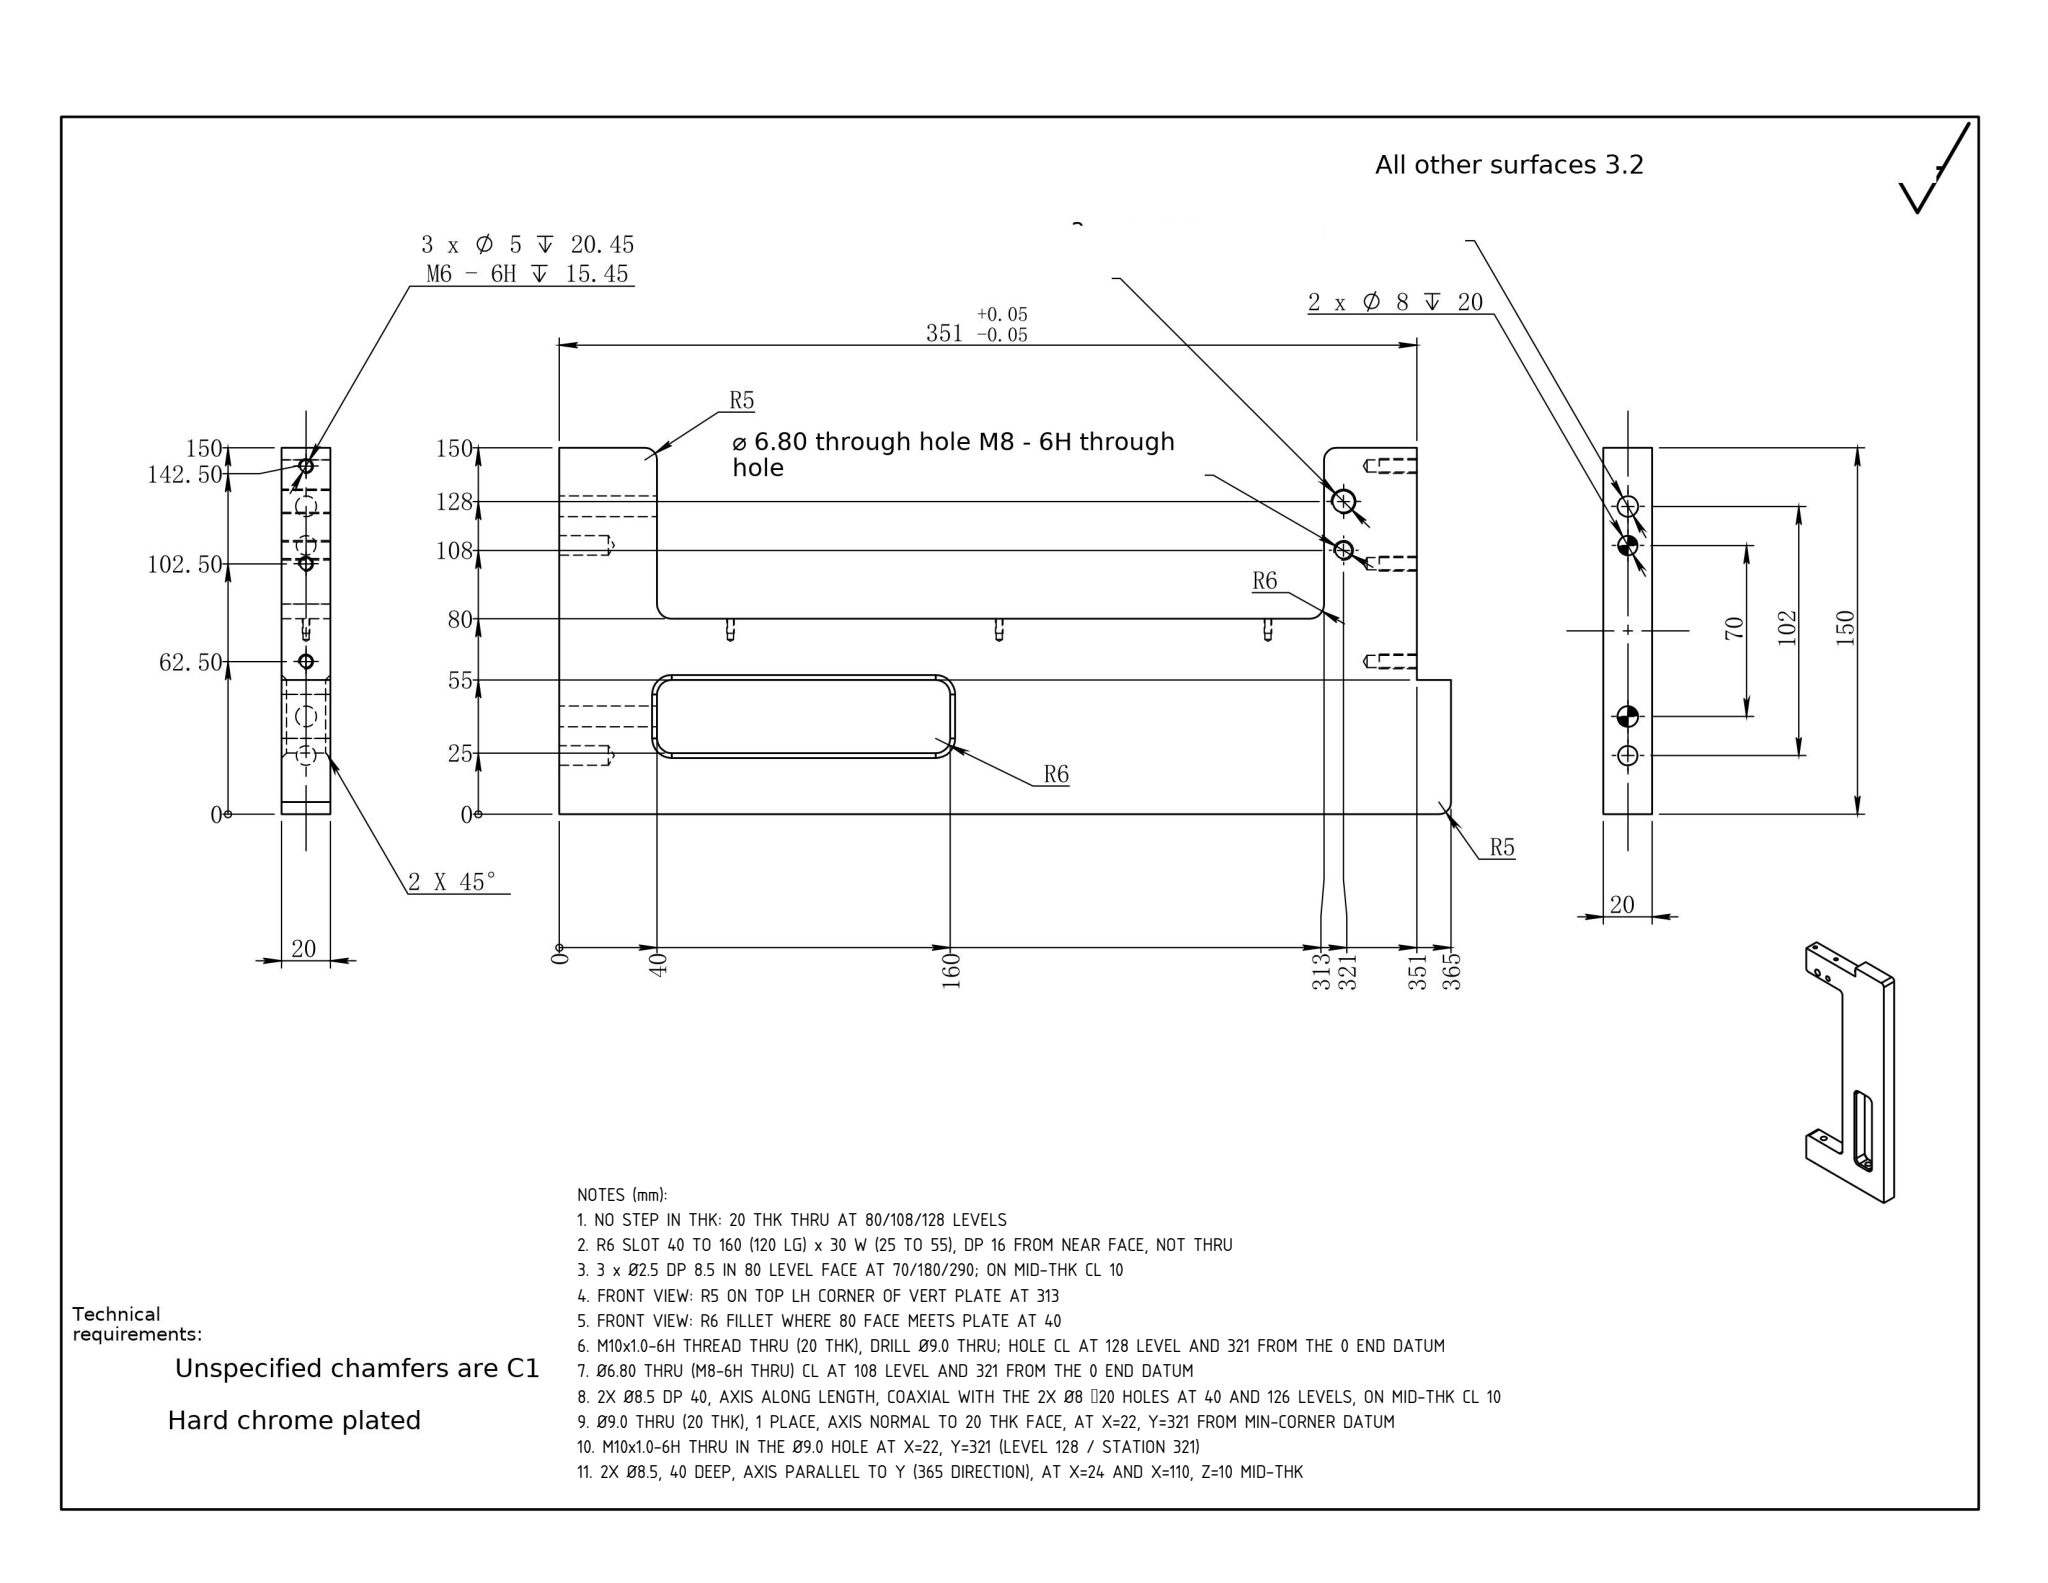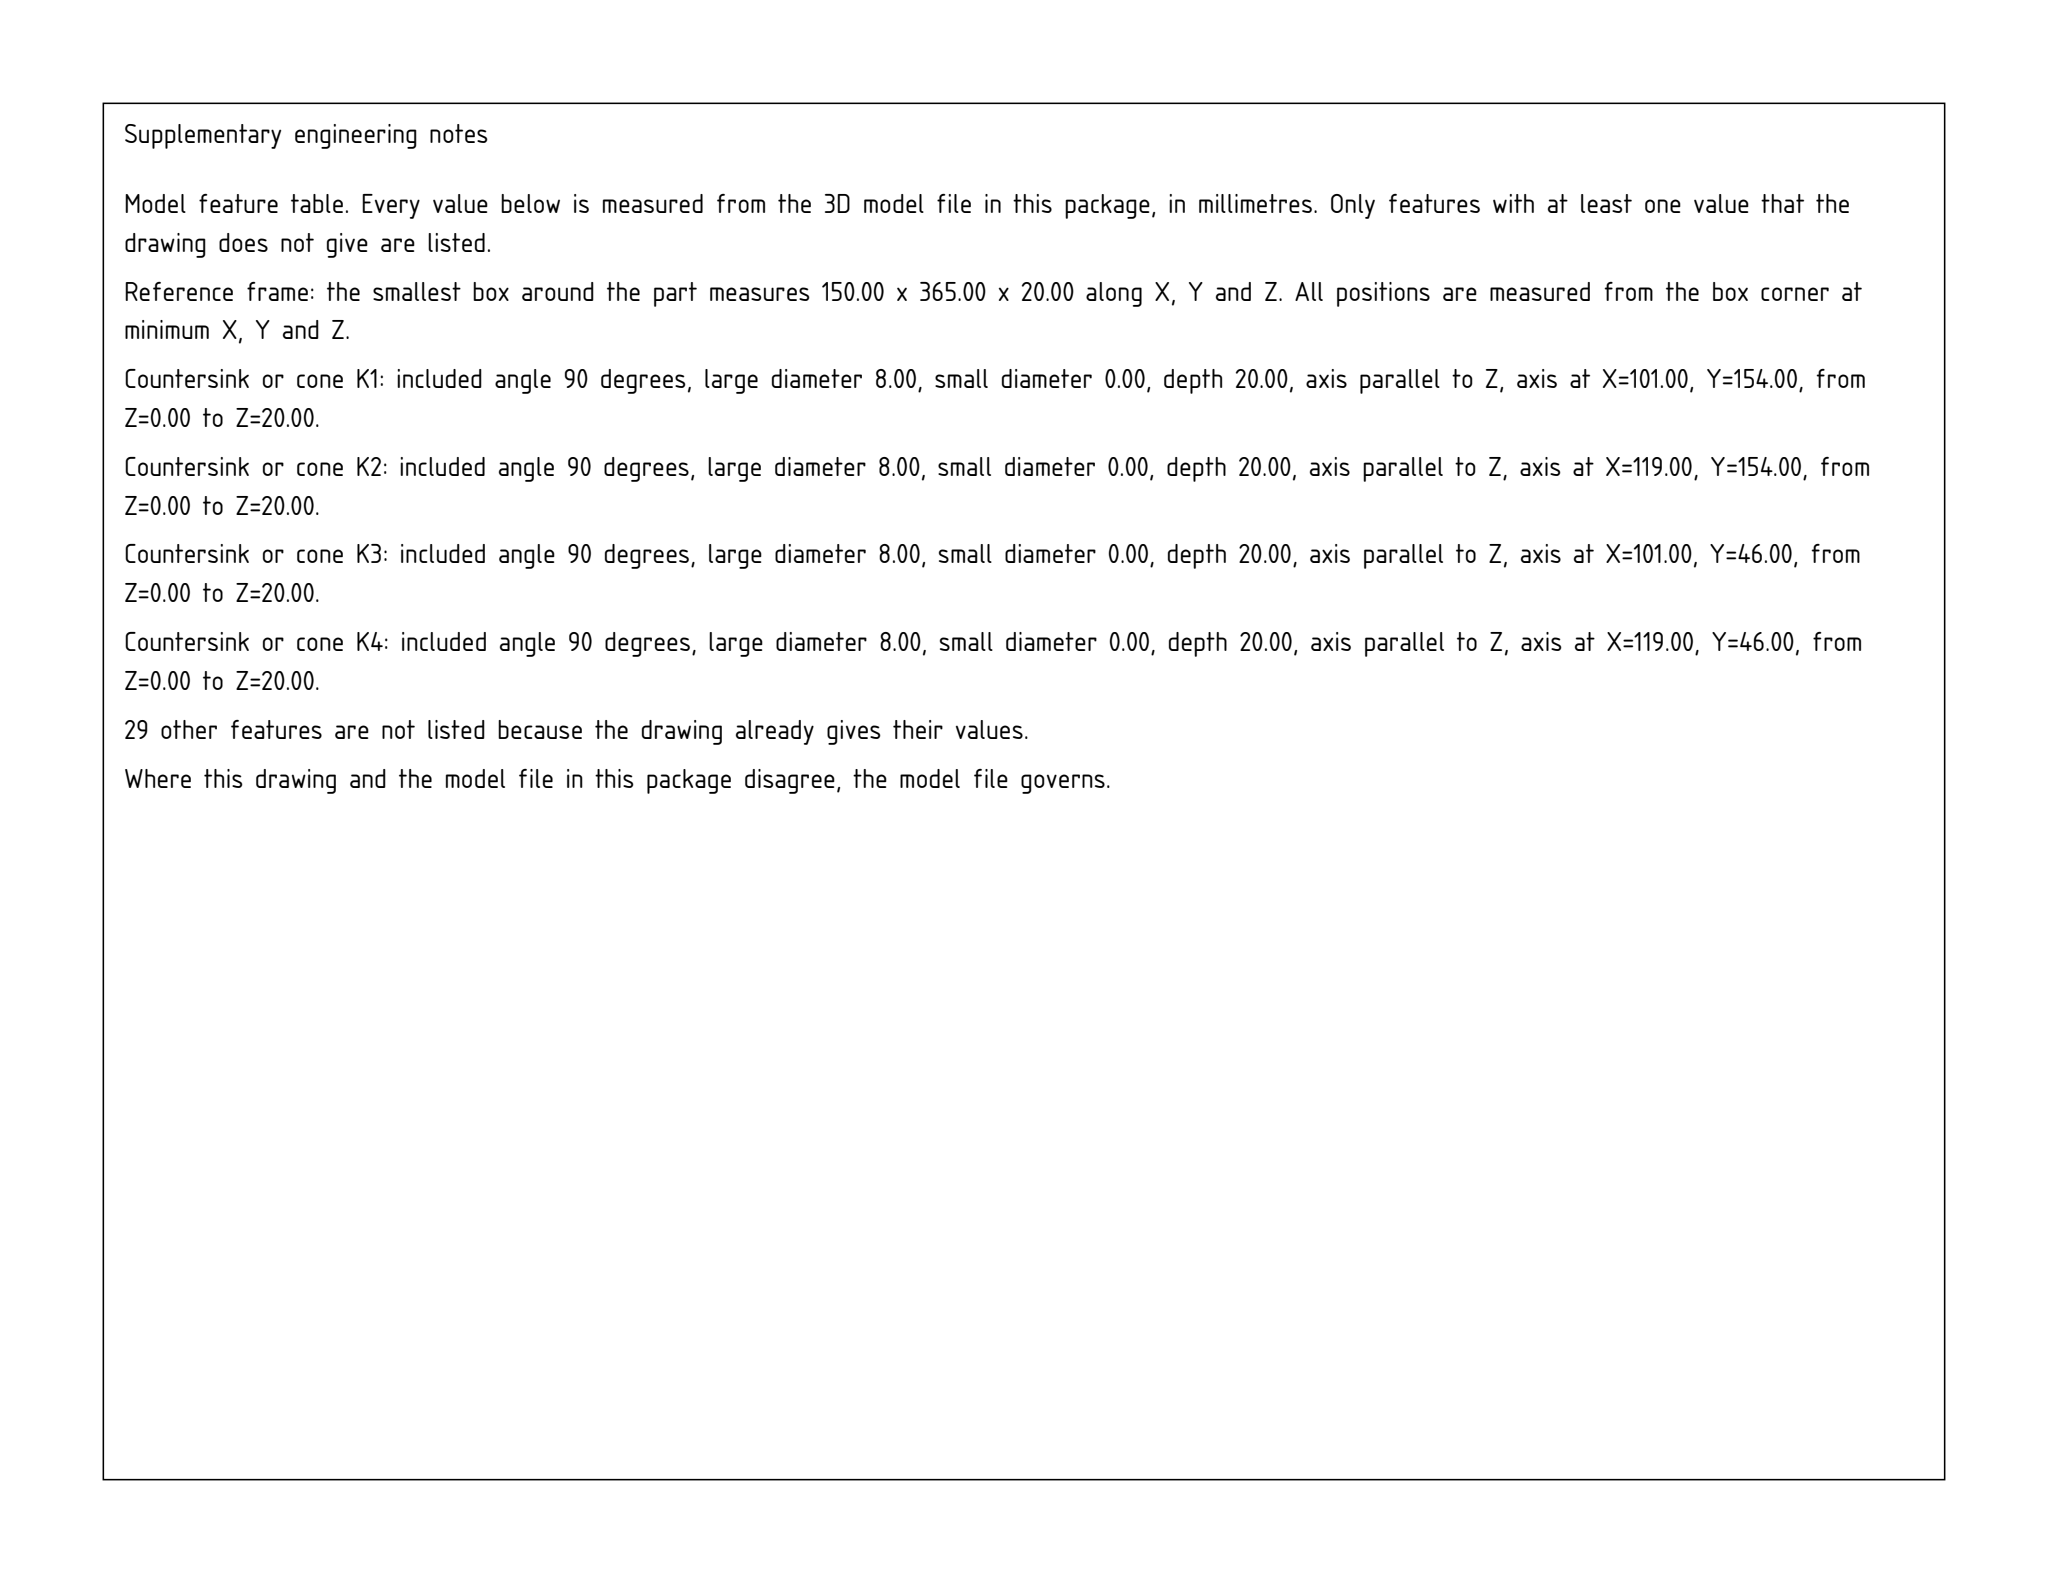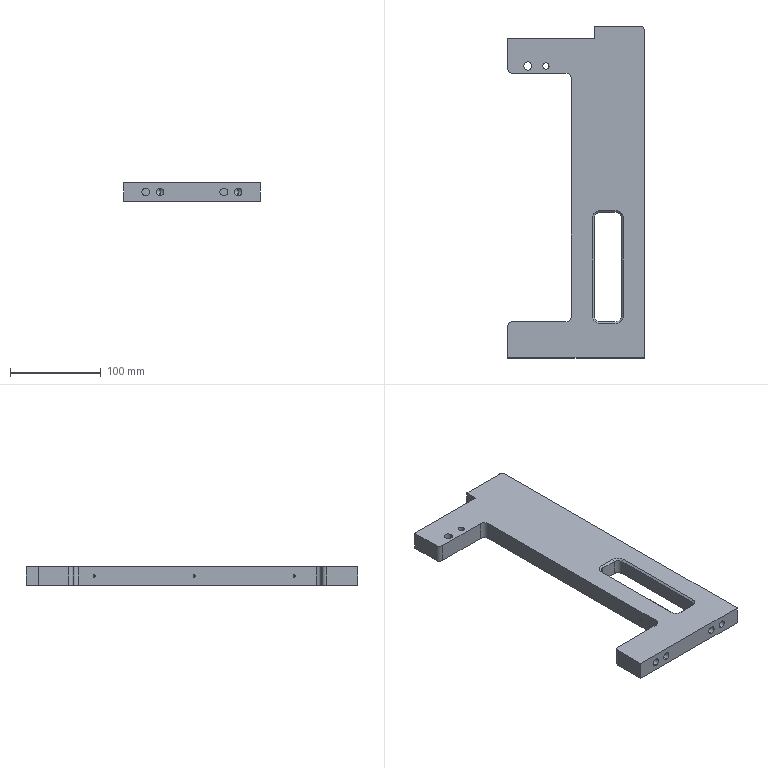Part | SolidWorks | mm | 1 solid | 81 faces | box 150 x 365 x 20 mm | volume 603637 mm3 | cylinder 33 | cone 24 | plane 24 | commonest cylinder face diameters 2.5 x6 5 x6 12 x6 8 x4 8.5 x4 10 x3 6.8 x2 9 x2
Drawing notes:
NO STEP IN THK: 20 THK THRU AT 80/108/128 LEVELS | from the solid: only z planes 0 and 20; Ø12 R6 corner cyls at x=64 len 20 (thru) at 80 level; 108/128 are Ø6.8 and Ø9 thru holes at y=321
R6 SLOT 40 TO 160 (120 LG) x 30 W (25 TO 55), DP 16 FROM NEAR FACE, NOT THRU | from the solid: Ø12 z-axis corner cyls at x=101/119, y=46/154 -> slot y 40-160, x 95-125 (25-55 from bottom); cyl length 16 vs 20 thk
3 x Ø2.5 DP 8.5 IN 80 LEVEL FACE AT 70/180/290; ON MID-THK CL 10 | from the solid: cylinders Ø2.5 axis x, length 8.5, pos [null,70/180/290,10], drilled from x=80 face; bbox z=20
FRONT VIEW: R5 ON TOP LH CORNER OF VERT PLATE AT 313 | from the solid: Vertical plate bounded by y-planes 313/351, top face z=150; corner round R5 at y=313, z=150 (bbox 150x365x20)
FRONT VIEW: R6 FILLET WHERE 80 FACE MEETS PLATE AT 40 | from the solid: Horizontal face z=80 meets y=40 plate face; internal fillet R6 (y-planes 0/40, z-level 80)
M10x1.0-6H THREAD THRU (20 THK), DRILL Ø9.0 THRU; HOLE CL AT 128 LEVEL AND 321 FROM THE 0 END DATUM | from the solid: cylinder dia 9.0, axis z, pos [x=22.0 (=150-128 level), y=321.0], length 20.0
Ø6.80 THRU (M8-6H THRU) CL AT 108 LEVEL AND 321 FROM THE 0 END DATUM | from the solid: cylinder dia 6.8, axis z, pos [x=42.0 (=150-108 level), y=321.0], length 20.0
2X Ø8.5 DP 40, AXIS ALONG LENGTH, COAXIAL WITH THE 2X Ø8 ⍈20 HOLES AT 40 AND 126 LEVELS, ON MID-THK CL 10 | from the solid: cylinders dia 8.5, axis y, pos [x=24.0 (=126 level), z=10.0] and [x=110.0 (=40 level), z=10.0], length 40.0
Ø9.0 THRU (20 THK), 1 PLACE, AXIS NORMAL TO 20 THK FACE, AT X=22, Y=321 FROM MIN-CORNER DATUM | from the solid: cylinders: [9.0,"z",[22.0,321.0,null],20.0]
M10x1.0-6H THRU IN THE Ø9.0 HOLE AT X=22, Y=321 (LEVEL 128 / STATION 321) | from the solid: cylinders: [9.0,"z",[22.0,321.0,null],20.0] = M10x1.0 tap drill; z-plane 0.0/20.0 THRU
2X Ø8.5, 40 DEEP, AXIS PARALLEL TO Y (365 DIRECTION), AT X=24 AND X=110, Z=10 MID-THK | from the solid: cylinders: [8.5,"y",[24.0,null,10.0],40.0] and [8.5,"y",[110.0,null,10.0],40.0]
build123d program:
from build123d import *

# Parameters (mm, degrees)
SKETCH1_W                      = 150
SKETCH1_H                      = 20
BOSS_EXTRUDE1_DEPTH            = 365
SKETCH2_W                      = 70
SKETCH2_H                      = 273
CUT_EXTRUDE1_DEPTH             = 374.162
CUT_EXTRUDE2_DEPTH             = 374.162
CUT_EXTRUDE2_DEPTH_BACK        = 374.162
SKETCH3_W                      = 95
SKETCH3_H                      = 14
CUT_EXTRUDE3_DEPTH             = 374.162
CUT_EXTRUDE3_DEPTH_BACK        = 374.162
SKETCH4_W                      = 30
SKETCH4_H                      = 120
FILLET1_R                      = 6
M10X1_0_TAPPED_HOLE1_D         = 9
M8_TAPPED_HOLE1_D              = 6.8
F_8_5_8_5_DIAMETER_HOLE1_D     = 8.5
F_8_5_8_5_DIAMETER_HOLE1_DEPTH = 40
F_8_0_8_DIAMETER_HOLE1_D       = 8
F_8_0_8_DIAMETER_HOLE1_DEPTH   = 20
F_8_0_8_DIAMETER_HOLE1_TIP     = 2.403
M6_TAPPED_HOLE1_D              = 5
M6_TAPPED_HOLE1_DEPTH          = 20.45
M6_TAPPED_HOLE1_TIP            = 1.502
FILLET2_R                      = 5
CHAMFER1_SIZE                  = 2
LPATTERN1_COUNT                = 3
LPATTERN1_PITCH                = 110


with BuildPart() as part:
    # Sketch1 → Boss-Extrude1 (new body)
    with BuildSketch(Plane(origin=(0, 0, 0), x_dir=(1, 0, 0), z_dir=(0, 1, 0))):
        Rectangle(SKETCH1_W, SKETCH1_H)
    extrude(amount=BOSS_EXTRUDE1_DEPTH)

    # Sketch2 → Cut-Extrude1 (cut, through all)
    with BuildSketch(Plane.XY.offset(10)):
        with Locations((-40, 176.5)):
            Rectangle(SKETCH2_W, SKETCH2_H)
    extrude(amount=-CUT_EXTRUDE1_DEPTH, mode=Mode.SUBTRACT)

    # Sketch3 → Cut-Extrude2 (cut, two sides: drawn at the far end of the back side and taken through both)
    with BuildSketch(Plane.XY.offset(10).offset(-CUT_EXTRUDE2_DEPTH_BACK)):
        with Locations((-27.5, 358)):
            Rectangle(SKETCH3_W, SKETCH3_H)
    extrude(amount=CUT_EXTRUDE2_DEPTH + CUT_EXTRUDE2_DEPTH_BACK, mode=Mode.SUBTRACT)

    # Sketch4 → Cut-Extrude3 (cut, two sides: drawn at the far end of the back side and taken through both)
    with BuildSketch(Plane.XY.offset(10).offset(-CUT_EXTRUDE3_DEPTH_BACK)):
        with Locations((35, 100)):
            Rectangle(SKETCH4_W, SKETCH4_H)
    extrude(amount=CUT_EXTRUDE3_DEPTH + CUT_EXTRUDE3_DEPTH_BACK, mode=Mode.SUBTRACT)

    # Fillet1
    fillet1_edges = [part.edges().sort_by_distance(p)[0] for p in [
        (-5, 313, 0),
        (-5, 40, 0),
        (50, 160, 0),
        (50, 40, 0),
        (20, 40, 0),
        (20, 160, 0),
    ]]
    fillet(fillet1_edges, radius=FILLET1_R)

    # M10x1.0 Tapped Hole1 (through all)
    with Locations(Plane.XY.offset(10)):
        with Locations((-53, 321)):
            Hole(M10X1_0_TAPPED_HOLE1_D / 2)

    # M8 Tapped Hole1 (through all)
    with Locations(Plane.XY.offset(10)):
        with Locations((-33, 321)):
            Hole(M8_TAPPED_HOLE1_D / 2)

    # 8.5 _8.5_ Diameter Hole1
    with Locations(Plane(origin=(0, 40, 0), x_dir=(1, 0, 0), z_dir=(0, 1, 0))):
        with Locations((-51, 0), (35, 0)):
            Hole(F_8_5_8_5_DIAMETER_HOLE1_D / 2, depth=F_8_5_8_5_DIAMETER_HOLE1_DEPTH)

    # 8.0 _8_ Diameter Hole1
    with Locations(Plane(origin=(0, 0, 0), x_dir=(-1, 0, 0), z_dir=(0, -1, 0))):
        with Locations((35, 0), (-51, 0)):
            Hole(F_8_0_8_DIAMETER_HOLE1_D / 2, depth=F_8_0_8_DIAMETER_HOLE1_DEPTH)
            with Locations((0, 0, -(F_8_0_8_DIAMETER_HOLE1_DEPTH + F_8_0_8_DIAMETER_HOLE1_TIP / 2))):  # 118° drill point
                Cone(0, F_8_0_8_DIAMETER_HOLE1_D / 2, F_8_0_8_DIAMETER_HOLE1_TIP, mode=Mode.SUBTRACT)

    # M6 Tapped Hole1
    with Locations(Plane(origin=(0, 351, 0), x_dir=(1, 0, 0), z_dir=(0, 1, 0))):
        with Locations((-67.5, 0), (12.5, 0), (-27.5, 0)):
            Hole(M6_TAPPED_HOLE1_D / 2, depth=M6_TAPPED_HOLE1_DEPTH)
            with Locations((0, 0, -(M6_TAPPED_HOLE1_DEPTH + M6_TAPPED_HOLE1_TIP / 2))):  # 118° drill point
                Cone(0, M6_TAPPED_HOLE1_D / 2, M6_TAPPED_HOLE1_TIP, mode=Mode.SUBTRACT)

    # Fillet2
    fillet2_edges = [part.edges().sort_by_distance(p)[0] for p in [
        (-75, 40, 0),
        (-75, 313, 0),
        (75, 365, 0),
    ]]
    fillet(fillet2_edges, radius=FILLET2_R)

    # Chamfer1
    chamfer1_edges = [part.edges().sort_by_distance(p)[0] for p in [
        (50, 100, -10),
        (50, 100, 10),
        (35, 40, -10),
        (35, 40, 10),
        (20, 100, -10),
        (20, 100, 10),
        (35, 160, -10),
        (35, 160, 10),
        (48.243, 41.757, 10),
        (48.243, 41.757, -10),
        (21.757, 41.757, 10),
        (21.757, 41.757, -10),
        (48.243, 158.243, 10),
        (48.243, 158.243, -10),
        (21.757, 158.243, 10),
        (21.757, 158.243, -10),
    ]]
    chamfer(chamfer1_edges, length=CHAMFER1_SIZE)

    # Sketch18 → M3 Tapped Hole1 (revolve, cut)
    with BuildSketch(Plane(origin=(-5, 290, 0), x_dir=(0, 0, 1), z_dir=(0, 1, 0))):
        Polygon((0, 0), (0, 9.251), (1.25, 8.5), (1.25, 0), align=None)
    m3_tapped_hole1 = revolve(axis=Axis((-11.35, 290, 0), (1, 0, 0)), mode=Mode.SUBTRACT)

    # LPattern1: M3 Tapped Hole1 ×3
    with Locations(*[(0, -i * LPATTERN1_PITCH, 0) for i in range(1, LPATTERN1_COUNT)]):
        add(m3_tapped_hole1, mode=Mode.SUBTRACT)


solid = part.part